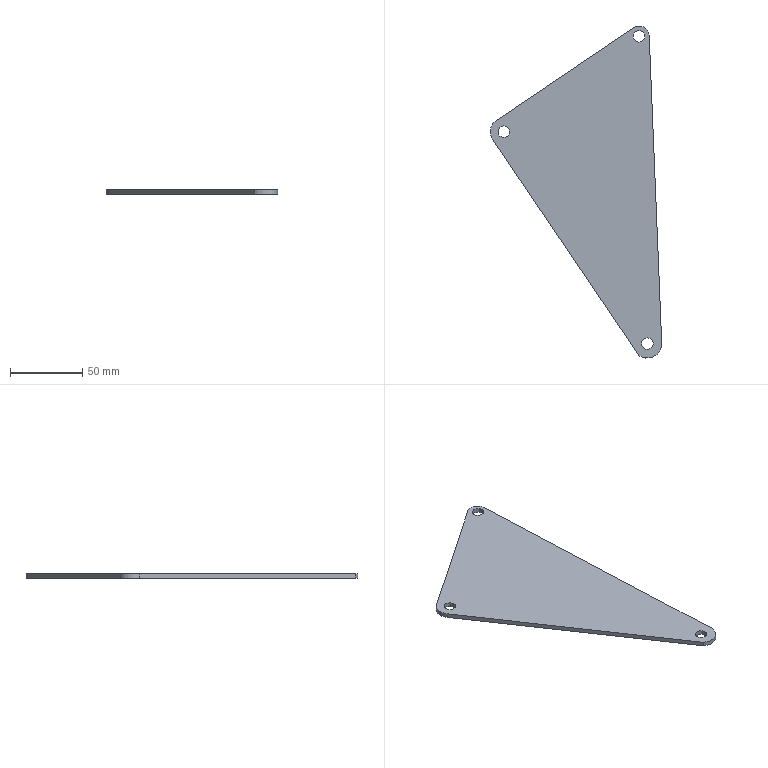Component | SolidWorks | gen par_a-2 | 1 solid | 15 faces | box 118.62 x 229.7 x 3 mm | volume 43932 mm3 | cylinder 10 | plane 5 | commonest cylinder face diameters 8 x6 14.196 x2 20 x1 18.711 x1
STEP:
#1=CARTESIAN_POINT('',(8.88,0.8832,7.243));
#2=VERTEX_POINT('',#1);
#3=CARTESIAN_POINT('',(9.14,1.06,7.243));
#4=VERTEX_POINT('',#3);
#5=CARTESIAN_POINT('',(9.01,0.9715,7.243));
#6=DIRECTION('',(-0.,0.,1.));
#7=DIRECTION('',(0.8279,0.5608,0.));
#8=AXIS2_PLACEMENT_3D('',#5,#6,#7);
#9=CIRCLE('',#8,0.1575);
#10=EDGE_CURVE('',#2,#4,#9,.T.);
#11=ORIENTED_EDGE('',*,*,#10,.F.);
#12=CARTESIAN_POINT('',(8.88,0.8832,7.361));
#13=VERTEX_POINT('',#12);
#14=CARTESIAN_POINT('',(8.88,0.8832,7.243));
#15=DIRECTION('',(-0.,0.,1.));
#16=VECTOR('',#15,39.37);
#17=LINE('',#14,#16);
#18=EDGE_CURVE('',#2,#13,#17,.T.);
#19=ORIENTED_EDGE('',*,*,#18,.T.);
#20=CARTESIAN_POINT('',(9.14,1.06,7.361));
#21=VERTEX_POINT('',#20);
#22=CARTESIAN_POINT('',(9.01,0.9715,7.361));
#23=DIRECTION('',(-0.,0.,1.));
#24=DIRECTION('',(0.8279,0.5608,0.));
#25=AXIS2_PLACEMENT_3D('',#22,#23,#24);
#26=CIRCLE('',#25,0.1575);
#27=EDGE_CURVE('',#13,#21,#26,.T.);
#28=ORIENTED_EDGE('',*,*,#27,.T.);
#29=CARTESIAN_POINT('',(9.14,1.06,7.243));
#30=DIRECTION('',(-0.,0.,1.));
#31=VECTOR('',#30,39.37);
#32=LINE('',#29,#31);
#33=EDGE_CURVE('',#4,#21,#32,.T.);
#34=ORIENTED_EDGE('',*,*,#33,.F.);
#35=EDGE_LOOP('',(#11,#19,#28,#34));
#36=FACE_OUTER_BOUND('',#35,.T.);
#37=CARTESIAN_POINT('',(9.01,0.9715,7.243));
#38=DIRECTION('',(-0.,0.,1.));
#39=DIRECTION('',(0.8279,0.5608,0.));
#40=AXIS2_PLACEMENT_3D('',#37,#38,#39);
#41=CYLINDRICAL_SURFACE('',#40,0.1575);
#42=ADVANCED_FACE('',(#36),#41,.F.);
#43=CARTESIAN_POINT('',(8.652,9.253,7.243));
#44=VERTEX_POINT('',#43);
#45=CARTESIAN_POINT('',(8.913,9.43,7.243));
#46=VERTEX_POINT('',#45);
#47=CARTESIAN_POINT('',(8.783,9.342,7.243));
#48=DIRECTION('',(-0.,0.,1.));
#49=DIRECTION('',(0.8279,0.5608,0.));
#50=AXIS2_PLACEMENT_3D('',#47,#48,#49);
#51=CIRCLE('',#50,0.1575);
#52=EDGE_CURVE('',#44,#46,#51,.T.);
#53=ORIENTED_EDGE('',*,*,#52,.F.);
#54=CARTESIAN_POINT('',(8.652,9.253,7.361));
#55=VERTEX_POINT('',#54);
#56=CARTESIAN_POINT('',(8.652,9.253,7.243));
#57=DIRECTION('',(-0.,0.,1.));
#58=VECTOR('',#57,39.37);
#59=LINE('',#56,#58);
#60=EDGE_CURVE('',#44,#55,#59,.T.);
#61=ORIENTED_EDGE('',*,*,#60,.T.);
#62=CARTESIAN_POINT('',(8.913,9.43,7.361));
#63=VERTEX_POINT('',#62);
#64=CARTESIAN_POINT('',(8.783,9.342,7.361));
#65=DIRECTION('',(-0.,0.,1.));
#66=DIRECTION('',(0.8279,0.5608,0.));
#67=AXIS2_PLACEMENT_3D('',#64,#65,#66);
#68=CIRCLE('',#67,0.1575);
#69=EDGE_CURVE('',#55,#63,#68,.T.);
#70=ORIENTED_EDGE('',*,*,#69,.T.);
#71=CARTESIAN_POINT('',(8.913,9.43,7.243));
#72=DIRECTION('',(-0.,0.,1.));
#73=VECTOR('',#72,39.37);
#74=LINE('',#71,#73);
#75=EDGE_CURVE('',#46,#63,#74,.T.);
#76=ORIENTED_EDGE('',*,*,#75,.F.);
#77=EDGE_LOOP('',(#53,#61,#70,#76));
#78=FACE_OUTER_BOUND('',#77,.T.);
#79=CARTESIAN_POINT('',(8.783,9.342,7.243));
#80=DIRECTION('',(-0.,0.,1.));
#81=DIRECTION('',(0.8279,0.5608,0.));
#82=AXIS2_PLACEMENT_3D('',#79,#80,#81);
#83=CYLINDRICAL_SURFACE('',#82,0.1575);
#84=ADVANCED_FACE('',(#78),#83,.F.);
#85=CARTESIAN_POINT('',(4.971,6.653,7.243));
#86=VERTEX_POINT('',#85);
#87=CARTESIAN_POINT('',(5.232,6.829,7.243));
#88=VERTEX_POINT('',#87);
#89=CARTESIAN_POINT('',(5.102,6.741,7.243));
#90=DIRECTION('',(-0.,0.,1.));
#91=DIRECTION('',(0.8279,0.5608,0.));
#92=AXIS2_PLACEMENT_3D('',#89,#90,#91);
#93=CIRCLE('',#92,0.1575);
#94=EDGE_CURVE('',#86,#88,#93,.T.);
#95=ORIENTED_EDGE('',*,*,#94,.F.);
#96=CARTESIAN_POINT('',(4.971,6.653,7.361));
#97=VERTEX_POINT('',#96);
#98=CARTESIAN_POINT('',(4.971,6.653,7.243));
#99=DIRECTION('',(-0.,0.,1.));
#100=VECTOR('',#99,39.37);
#101=LINE('',#98,#100);
#102=EDGE_CURVE('',#86,#97,#101,.T.);
#103=ORIENTED_EDGE('',*,*,#102,.T.);
#104=CARTESIAN_POINT('',(5.232,6.829,7.361));
#105=VERTEX_POINT('',#104);
#106=CARTESIAN_POINT('',(5.102,6.741,7.361));
#107=DIRECTION('',(-0.,0.,1.));
#108=DIRECTION('',(0.8279,0.5608,0.));
#109=AXIS2_PLACEMENT_3D('',#106,#107,#108);
#110=CIRCLE('',#109,0.1575);
#111=EDGE_CURVE('',#97,#105,#110,.T.);
#112=ORIENTED_EDGE('',*,*,#111,.T.);
#113=CARTESIAN_POINT('',(5.232,6.829,7.243));
#114=DIRECTION('',(-0.,0.,1.));
#115=VECTOR('',#114,39.37);
#116=LINE('',#113,#115);
#117=EDGE_CURVE('',#88,#105,#116,.T.);
#118=ORIENTED_EDGE('',*,*,#117,.F.);
#119=EDGE_LOOP('',(#95,#103,#112,#118));
#120=FACE_OUTER_BOUND('',#119,.T.);
#121=CARTESIAN_POINT('',(5.102,6.741,7.243));
#122=DIRECTION('',(-0.,0.,1.));
#123=DIRECTION('',(0.8279,0.5608,0.));
#124=AXIS2_PLACEMENT_3D('',#121,#122,#123);
#125=CYLINDRICAL_SURFACE('',#124,0.1575);
#126=ADVANCED_FACE('',(#120),#125,.F.);
#127=CARTESIAN_POINT('',(9.062,9.353,7.243));
#128=VERTEX_POINT('',#127);
#129=CARTESIAN_POINT('',(9.014,9.498,7.243));
#130=VERTEX_POINT('',#129);
#131=CARTESIAN_POINT('',(8.783,9.342,7.243));
#132=DIRECTION('',(-0.,0.,1.));
#133=DIRECTION('',(0.8279,0.5608,0.));
#134=AXIS2_PLACEMENT_3D('',#131,#132,#133);
#135=CIRCLE('',#134,0.2795);
#136=EDGE_CURVE('',#128,#130,#135,.T.);
#137=ORIENTED_EDGE('',*,*,#136,.T.);
#138=CARTESIAN_POINT('',(9.014,9.498,7.361));
#139=VERTEX_POINT('',#138);
#140=CARTESIAN_POINT('',(9.014,9.498,7.243));
#141=DIRECTION('',(-0.,0.,1.));
#142=VECTOR('',#141,39.37);
#143=LINE('',#140,#142);
#144=EDGE_CURVE('',#130,#139,#143,.T.);
#145=ORIENTED_EDGE('',*,*,#144,.T.);
#146=CARTESIAN_POINT('',(9.062,9.353,7.361));
#147=VERTEX_POINT('',#146);
#148=CARTESIAN_POINT('',(8.783,9.342,7.361));
#149=DIRECTION('',(-0.,0.,1.));
#150=DIRECTION('',(0.8279,0.5608,0.));
#151=AXIS2_PLACEMENT_3D('',#148,#149,#150);
#152=CIRCLE('',#151,0.2795);
#153=EDGE_CURVE('',#147,#139,#152,.T.);
#154=ORIENTED_EDGE('',*,*,#153,.F.);
#155=CARTESIAN_POINT('',(9.062,9.353,7.243));
#156=DIRECTION('',(-0.,0.,1.));
#157=VECTOR('',#156,39.37);
#158=LINE('',#155,#157);
#159=EDGE_CURVE('',#128,#147,#158,.T.);
#160=ORIENTED_EDGE('',*,*,#159,.F.);
#161=EDGE_LOOP('',(#137,#145,#154,#160));
#162=FACE_OUTER_BOUND('',#161,.T.);
#163=CARTESIAN_POINT('',(8.783,9.342,7.243));
#164=DIRECTION('',(-0.,0.,1.));
#165=DIRECTION('',(0.8279,0.5608,0.));
#166=AXIS2_PLACEMENT_3D('',#163,#164,#165);
#167=CYLINDRICAL_SURFACE('',#166,0.2795);
#168=ADVANCED_FACE('',(#162),#167,.T.);
#169=CARTESIAN_POINT('',(8.783,0.6498,7.361));
#170=VERTEX_POINT('',#169);
#171=CARTESIAN_POINT('',(9.403,0.9876,7.361));
#172=VERTEX_POINT('',#171);
#173=CARTESIAN_POINT('',(9.01,0.9715,7.361));
#174=DIRECTION('',(-0.,0.,1.));
#175=DIRECTION('',(0.8279,0.5608,0.));
#176=AXIS2_PLACEMENT_3D('',#173,#174,#175);
#177=CIRCLE('',#176,0.3937);
#178=EDGE_CURVE('',#170,#172,#177,.T.);
#179=ORIENTED_EDGE('',*,*,#178,.F.);
#180=CARTESIAN_POINT('',(8.783,0.6498,7.243));
#181=VERTEX_POINT('',#180);
#182=CARTESIAN_POINT('',(8.783,0.6498,7.243));
#183=DIRECTION('',(-0.,0.,1.));
#184=VECTOR('',#183,39.37);
#185=LINE('',#182,#184);
#186=EDGE_CURVE('',#181,#170,#185,.T.);
#187=ORIENTED_EDGE('',*,*,#186,.F.);
#188=CARTESIAN_POINT('',(9.403,0.9876,7.243));
#189=VERTEX_POINT('',#188);
#190=CARTESIAN_POINT('',(9.01,0.9715,7.243));
#191=DIRECTION('',(-0.,0.,1.));
#192=DIRECTION('',(0.8279,0.5608,0.));
#193=AXIS2_PLACEMENT_3D('',#190,#191,#192);
#194=CIRCLE('',#193,0.3937);
#195=EDGE_CURVE('',#181,#189,#194,.T.);
#196=ORIENTED_EDGE('',*,*,#195,.T.);
#197=CARTESIAN_POINT('',(9.403,0.9876,7.243));
#198=DIRECTION('',(-0.,0.,1.));
#199=VECTOR('',#198,39.37);
#200=LINE('',#197,#199);
#201=EDGE_CURVE('',#189,#172,#200,.T.);
#202=ORIENTED_EDGE('',*,*,#201,.T.);
#203=EDGE_LOOP('',(#179,#187,#196,#202));
#204=FACE_OUTER_BOUND('',#203,.T.);
#205=CARTESIAN_POINT('',(9.01,0.9715,7.243));
#206=DIRECTION('',(-0.,0.,1.));
#207=DIRECTION('',(0.8279,0.5608,0.));
#208=AXIS2_PLACEMENT_3D('',#205,#206,#207);
#209=CYLINDRICAL_SURFACE('',#208,0.3937);
#210=ADVANCED_FACE('',(#204),#209,.T.);
#211=CARTESIAN_POINT('',(4.797,6.534,7.361));
#212=VERTEX_POINT('',#211);
#213=CARTESIAN_POINT('',(8.783,0.6498,7.361));
#214=DIRECTION('',(0.5608,-0.8279,0.));
#215=VECTOR('',#214,39.37);
#216=LINE('',#213,#215);
#217=EDGE_CURVE('',#212,#170,#216,.T.);
#218=ORIENTED_EDGE('',*,*,#217,.F.);
#219=CARTESIAN_POINT('',(4.797,6.534,7.243));
#220=VERTEX_POINT('',#219);
#221=CARTESIAN_POINT('',(4.797,6.534,7.243));
#222=DIRECTION('',(-0.,0.,1.));
#223=VECTOR('',#222,39.37);
#224=LINE('',#221,#223);
#225=EDGE_CURVE('',#220,#212,#224,.T.);
#226=ORIENTED_EDGE('',*,*,#225,.F.);
#227=CARTESIAN_POINT('',(8.783,0.6498,7.243));
#228=DIRECTION('',(0.5608,-0.8279,0.));
#229=VECTOR('',#228,39.37);
#230=LINE('',#227,#229);
#231=EDGE_CURVE('',#220,#181,#230,.T.);
#232=ORIENTED_EDGE('',*,*,#231,.T.);
#233=ORIENTED_EDGE('',*,*,#186,.T.);
#234=EDGE_LOOP('',(#218,#226,#232,#233));
#235=FACE_OUTER_BOUND('',#234,.T.);
#236=CARTESIAN_POINT('',(8.783,0.6498,7.243));
#237=DIRECTION('',(-0.8279,-0.5608,-0.));
#238=DIRECTION('',(-0.,0.,1.));
#239=AXIS2_PLACEMENT_3D('',#236,#237,#238);
#240=PLANE('',#239);
#241=ADVANCED_FACE('',(#235),#240,.T.);
#242=CARTESIAN_POINT('',(4.895,7.046,7.361));
#243=VERTEX_POINT('',#242);
#244=CARTESIAN_POINT('',(5.102,6.741,7.361));
#245=DIRECTION('',(-0.,0.,1.));
#246=DIRECTION('',(-0.8279,-0.5608,0.));
#247=AXIS2_PLACEMENT_3D('',#244,#245,#246);
#248=CIRCLE('',#247,0.3683);
#249=EDGE_CURVE('',#243,#212,#248,.T.);
#250=ORIENTED_EDGE('',*,*,#249,.F.);
#251=CARTESIAN_POINT('',(4.895,7.046,7.243));
#252=VERTEX_POINT('',#251);
#253=CARTESIAN_POINT('',(4.895,7.046,7.243));
#254=DIRECTION('',(-0.,0.,1.));
#255=VECTOR('',#254,39.37);
#256=LINE('',#253,#255);
#257=EDGE_CURVE('',#252,#243,#256,.T.);
#258=ORIENTED_EDGE('',*,*,#257,.F.);
#259=CARTESIAN_POINT('',(5.102,6.741,7.243));
#260=DIRECTION('',(-0.,0.,1.));
#261=DIRECTION('',(-0.8279,-0.5608,0.));
#262=AXIS2_PLACEMENT_3D('',#259,#260,#261);
#263=CIRCLE('',#262,0.3683);
#264=EDGE_CURVE('',#252,#220,#263,.T.);
#265=ORIENTED_EDGE('',*,*,#264,.T.);
#266=ORIENTED_EDGE('',*,*,#225,.T.);
#267=EDGE_LOOP('',(#250,#258,#265,#266));
#268=FACE_OUTER_BOUND('',#267,.T.);
#269=CARTESIAN_POINT('',(5.102,6.741,7.243));
#270=DIRECTION('',(-0.,0.,1.));
#271=DIRECTION('',(0.8279,0.5608,0.));
#272=AXIS2_PLACEMENT_3D('',#269,#270,#271);
#273=CYLINDRICAL_SURFACE('',#272,0.3683);
#274=ADVANCED_FACE('',(#268),#273,.T.);
#275=CARTESIAN_POINT('',(8.626,9.573,7.361));
#276=VERTEX_POINT('',#275);
#277=CARTESIAN_POINT('',(4.895,7.046,7.361));
#278=DIRECTION('',(-0.8279,-0.5608,-0.));
#279=VECTOR('',#278,39.37);
#280=LINE('',#277,#279);
#281=EDGE_CURVE('',#276,#243,#280,.T.);
#282=ORIENTED_EDGE('',*,*,#281,.F.);
#283=CARTESIAN_POINT('',(8.626,9.573,7.243));
#284=VERTEX_POINT('',#283);
#285=CARTESIAN_POINT('',(8.626,9.573,7.243));
#286=DIRECTION('',(-0.,0.,1.));
#287=VECTOR('',#286,39.37);
#288=LINE('',#285,#287);
#289=EDGE_CURVE('',#284,#276,#288,.T.);
#290=ORIENTED_EDGE('',*,*,#289,.F.);
#291=CARTESIAN_POINT('',(4.895,7.046,7.243));
#292=DIRECTION('',(-0.8279,-0.5608,-0.));
#293=VECTOR('',#292,39.37);
#294=LINE('',#291,#293);
#295=EDGE_CURVE('',#284,#252,#294,.T.);
#296=ORIENTED_EDGE('',*,*,#295,.T.);
#297=ORIENTED_EDGE('',*,*,#257,.T.);
#298=EDGE_LOOP('',(#282,#290,#296,#297));
#299=FACE_OUTER_BOUND('',#298,.T.);
#300=CARTESIAN_POINT('',(4.895,7.046,7.243));
#301=DIRECTION('',(-0.5608,0.8279,-0.));
#302=DIRECTION('',(-0.8279,-0.5608,-0.));
#303=AXIS2_PLACEMENT_3D('',#300,#301,#302);
#304=PLANE('',#303);
#305=ADVANCED_FACE('',(#299),#304,.T.);
#306=ORIENTED_EDGE('',*,*,#144,.F.);
#307=CARTESIAN_POINT('',(8.783,9.342,7.243));
#308=DIRECTION('',(-0.,0.,1.));
#309=DIRECTION('',(0.8279,0.5608,0.));
#310=AXIS2_PLACEMENT_3D('',#307,#308,#309);
#311=CIRCLE('',#310,0.2795);
#312=EDGE_CURVE('',#130,#284,#311,.T.);
#313=ORIENTED_EDGE('',*,*,#312,.T.);
#314=ORIENTED_EDGE('',*,*,#289,.T.);
#315=CARTESIAN_POINT('',(8.783,9.342,7.361));
#316=DIRECTION('',(-0.,0.,1.));
#317=DIRECTION('',(0.8279,0.5608,0.));
#318=AXIS2_PLACEMENT_3D('',#315,#316,#317);
#319=CIRCLE('',#318,0.2795);
#320=EDGE_CURVE('',#139,#276,#319,.T.);
#321=ORIENTED_EDGE('',*,*,#320,.F.);
#322=EDGE_LOOP('',(#306,#313,#314,#321));
#323=FACE_OUTER_BOUND('',#322,.T.);
#324=CARTESIAN_POINT('',(8.783,9.342,7.243));
#325=DIRECTION('',(-0.,0.,1.));
#326=DIRECTION('',(0.8279,0.5608,0.));
#327=AXIS2_PLACEMENT_3D('',#324,#325,#326);
#328=CYLINDRICAL_SURFACE('',#327,0.2795);
#329=ADVANCED_FACE('',(#323),#328,.T.);
#330=CARTESIAN_POINT('',(9.403,0.9876,7.361));
#331=DIRECTION('',(-0.04078,0.9992,-0.));
#332=VECTOR('',#331,39.37);
#333=LINE('',#330,#332);
#334=EDGE_CURVE('',#172,#147,#333,.T.);
#335=ORIENTED_EDGE('',*,*,#334,.F.);
#336=ORIENTED_EDGE('',*,*,#201,.F.);
#337=CARTESIAN_POINT('',(9.403,0.9876,7.243));
#338=DIRECTION('',(-0.04078,0.9992,-0.));
#339=VECTOR('',#338,39.37);
#340=LINE('',#337,#339);
#341=EDGE_CURVE('',#189,#128,#340,.T.);
#342=ORIENTED_EDGE('',*,*,#341,.T.);
#343=ORIENTED_EDGE('',*,*,#159,.T.);
#344=EDGE_LOOP('',(#335,#336,#342,#343));
#345=FACE_OUTER_BOUND('',#344,.T.);
#346=CARTESIAN_POINT('',(9.403,0.9876,7.243));
#347=DIRECTION('',(0.9992,0.04078,0.));
#348=DIRECTION('',(-0.04078,0.9992,-0.));
#349=AXIS2_PLACEMENT_3D('',#346,#347,#348);
#350=PLANE('',#349);
#351=ADVANCED_FACE('',(#345),#350,.T.);
#352=CARTESIAN_POINT('',(9.01,0.9715,7.243));
#353=DIRECTION('',(-0.,0.,1.));
#354=DIRECTION('',(0.8279,0.5608,0.));
#355=AXIS2_PLACEMENT_3D('',#352,#353,#354);
#356=CIRCLE('',#355,0.1575);
#357=EDGE_CURVE('',#4,#2,#356,.T.);
#358=ORIENTED_EDGE('',*,*,#357,.T.);
#359=ORIENTED_EDGE('',*,*,#10,.T.);
#360=EDGE_LOOP('',(#358,#359));
#361=FACE_BOUND('',#360,.T.);
#362=CARTESIAN_POINT('',(8.783,9.342,7.243));
#363=DIRECTION('',(-0.,0.,1.));
#364=DIRECTION('',(0.8279,0.5608,0.));
#365=AXIS2_PLACEMENT_3D('',#362,#363,#364);
#366=CIRCLE('',#365,0.1575);
#367=EDGE_CURVE('',#46,#44,#366,.T.);
#368=ORIENTED_EDGE('',*,*,#367,.T.);
#369=ORIENTED_EDGE('',*,*,#52,.T.);
#370=EDGE_LOOP('',(#368,#369));
#371=FACE_BOUND('',#370,.T.);
#372=CARTESIAN_POINT('',(5.102,6.741,7.243));
#373=DIRECTION('',(-0.,0.,1.));
#374=DIRECTION('',(0.8279,0.5608,0.));
#375=AXIS2_PLACEMENT_3D('',#372,#373,#374);
#376=CIRCLE('',#375,0.1575);
#377=EDGE_CURVE('',#88,#86,#376,.T.);
#378=ORIENTED_EDGE('',*,*,#377,.T.);
#379=ORIENTED_EDGE('',*,*,#94,.T.);
#380=EDGE_LOOP('',(#378,#379));
#381=FACE_BOUND('',#380,.T.);
#382=ORIENTED_EDGE('',*,*,#195,.F.);
#383=ORIENTED_EDGE('',*,*,#231,.F.);
#384=ORIENTED_EDGE('',*,*,#264,.F.);
#385=ORIENTED_EDGE('',*,*,#295,.F.);
#386=ORIENTED_EDGE('',*,*,#312,.F.);
#387=ORIENTED_EDGE('',*,*,#136,.F.);
#388=ORIENTED_EDGE('',*,*,#341,.F.);
#389=EDGE_LOOP('',(#382,#383,#384,#385,#386,#387,#388));
#390=FACE_OUTER_BOUND('',#389,.T.);
#391=CARTESIAN_POINT('',(9.01,0.9715,7.243));
#392=DIRECTION('',(-0.,0.,1.));
#393=DIRECTION('',(0.8279,0.5608,0.));
#394=AXIS2_PLACEMENT_3D('',#391,#392,#393);
#395=PLANE('',#394);
#396=ADVANCED_FACE('',(#361,#371,#381,#390),#395,.F.);
#397=CARTESIAN_POINT('',(9.01,0.9715,7.361));
#398=DIRECTION('',(-0.,0.,1.));
#399=DIRECTION('',(0.8279,0.5608,0.));
#400=AXIS2_PLACEMENT_3D('',#397,#398,#399);
#401=CIRCLE('',#400,0.1575);
#402=EDGE_CURVE('',#21,#13,#401,.T.);
#403=ORIENTED_EDGE('',*,*,#402,.F.);
#404=ORIENTED_EDGE('',*,*,#27,.F.);
#405=EDGE_LOOP('',(#403,#404));
#406=FACE_BOUND('',#405,.T.);
#407=CARTESIAN_POINT('',(8.783,9.342,7.361));
#408=DIRECTION('',(-0.,0.,1.));
#409=DIRECTION('',(0.8279,0.5608,0.));
#410=AXIS2_PLACEMENT_3D('',#407,#408,#409);
#411=CIRCLE('',#410,0.1575);
#412=EDGE_CURVE('',#63,#55,#411,.T.);
#413=ORIENTED_EDGE('',*,*,#412,.F.);
#414=ORIENTED_EDGE('',*,*,#69,.F.);
#415=EDGE_LOOP('',(#413,#414));
#416=FACE_BOUND('',#415,.T.);
#417=CARTESIAN_POINT('',(5.102,6.741,7.361));
#418=DIRECTION('',(-0.,0.,1.));
#419=DIRECTION('',(0.8279,0.5608,0.));
#420=AXIS2_PLACEMENT_3D('',#417,#418,#419);
#421=CIRCLE('',#420,0.1575);
#422=EDGE_CURVE('',#105,#97,#421,.T.);
#423=ORIENTED_EDGE('',*,*,#422,.F.);
#424=ORIENTED_EDGE('',*,*,#111,.F.);
#425=EDGE_LOOP('',(#423,#424));
#426=FACE_BOUND('',#425,.T.);
#427=ORIENTED_EDGE('',*,*,#178,.T.);
#428=ORIENTED_EDGE('',*,*,#334,.T.);
#429=ORIENTED_EDGE('',*,*,#153,.T.);
#430=ORIENTED_EDGE('',*,*,#320,.T.);
#431=ORIENTED_EDGE('',*,*,#281,.T.);
#432=ORIENTED_EDGE('',*,*,#249,.T.);
#433=ORIENTED_EDGE('',*,*,#217,.T.);
#434=EDGE_LOOP('',(#427,#428,#429,#430,#431,#432,#433));
#435=FACE_OUTER_BOUND('',#434,.T.);
#436=CARTESIAN_POINT('',(9.01,0.9715,7.361));
#437=DIRECTION('',(-0.,0.,1.));
#438=DIRECTION('',(0.8279,0.5608,0.));
#439=AXIS2_PLACEMENT_3D('',#436,#437,#438);
#440=PLANE('',#439);
#441=ADVANCED_FACE('',(#406,#416,#426,#435),#440,.T.);
#442=ORIENTED_EDGE('',*,*,#102,.F.);
#443=ORIENTED_EDGE('',*,*,#377,.F.);
#444=ORIENTED_EDGE('',*,*,#117,.T.);
#445=ORIENTED_EDGE('',*,*,#422,.T.);
#446=EDGE_LOOP('',(#442,#443,#444,#445));
#447=FACE_OUTER_BOUND('',#446,.T.);
#448=CARTESIAN_POINT('',(5.102,6.741,7.243));
#449=DIRECTION('',(-0.,0.,1.));
#450=DIRECTION('',(0.8279,0.5608,0.));
#451=AXIS2_PLACEMENT_3D('',#448,#449,#450);
#452=CYLINDRICAL_SURFACE('',#451,0.1575);
#453=ADVANCED_FACE('',(#447),#452,.F.);
#454=ORIENTED_EDGE('',*,*,#60,.F.);
#455=ORIENTED_EDGE('',*,*,#367,.F.);
#456=ORIENTED_EDGE('',*,*,#75,.T.);
#457=ORIENTED_EDGE('',*,*,#412,.T.);
#458=EDGE_LOOP('',(#454,#455,#456,#457));
#459=FACE_OUTER_BOUND('',#458,.T.);
#460=CARTESIAN_POINT('',(8.783,9.342,7.243));
#461=DIRECTION('',(-0.,0.,1.));
#462=DIRECTION('',(0.8279,0.5608,0.));
#463=AXIS2_PLACEMENT_3D('',#460,#461,#462);
#464=CYLINDRICAL_SURFACE('',#463,0.1575);
#465=ADVANCED_FACE('',(#459),#464,.F.);
#466=ORIENTED_EDGE('',*,*,#18,.F.);
#467=ORIENTED_EDGE('',*,*,#357,.F.);
#468=ORIENTED_EDGE('',*,*,#33,.T.);
#469=ORIENTED_EDGE('',*,*,#402,.T.);
#470=EDGE_LOOP('',(#466,#467,#468,#469));
#471=FACE_OUTER_BOUND('',#470,.T.);
#472=CARTESIAN_POINT('',(9.01,0.9715,7.243));
#473=DIRECTION('',(-0.,0.,1.));
#474=DIRECTION('',(0.8279,0.5608,0.));
#475=AXIS2_PLACEMENT_3D('',#472,#473,#474);
#476=CYLINDRICAL_SURFACE('',#475,0.1575);
#477=ADVANCED_FACE('',(#471),#476,.F.);
#478=CLOSED_SHELL('',(#42,#84,#126,#168,#210,#241,#274,#305,#329,#351,#396,#441,#453,#465,#477));
#479=MANIFOLD_SOLID_BREP('',#478);
#480=CARTESIAN_POINT('',(0.,0.,0.));
#481=DIRECTION('',(0.,0.,1.));
#482=DIRECTION('',(1.,0.,0.));
#483=AXIS2_PLACEMENT_3D('',#480,#481,#482);
#484=(LENGTH_UNIT()NAMED_UNIT(*)SI_UNIT($,.METRE.));
#485=LENGTH_MEASURE_WITH_UNIT(LENGTH_MEASURE(0.0254),#484);
#486=DIMENSIONAL_EXPONENTS(1.,0.,0.,0.,0.,0.,0.);
#487=(CONVERSION_BASED_UNIT('',#485)LENGTH_UNIT()NAMED_UNIT(#486));
#488=UNCERTAINTY_MEASURE_WITH_UNIT(LENGTH_MEASURE(0.00001),#487,'','');
#489=(NAMED_UNIT(*)PLANE_ANGLE_UNIT()SI_UNIT($,.RADIAN.));
#490=(NAMED_UNIT(*)SI_UNIT($,.STERADIAN.)SOLID_ANGLE_UNIT());
#491=(GEOMETRIC_REPRESENTATION_CONTEXT(3)GLOBAL_UNCERTAINTY_ASSIGNED_CONTEXT((#488))GLOBAL_UNIT_ASSIGNED_CONTEXT((#487,#489,#490))REPRESENTATION_CONTEXT('',''));
#492=ADVANCED_BREP_SHAPE_REPRESENTATION('',(#479,#483),#491);
#493=COLOUR_RGB('',0.7922,0.8196,0.9333);
#494=FILL_AREA_STYLE_COLOUR('',#493);
#495=FILL_AREA_STYLE('',(#494));
#496=SURFACE_STYLE_FILL_AREA(#495);
#497=SURFACE_SIDE_STYLE('',(#496));
#498=SURFACE_STYLE_USAGE(.BOTH.,#497);
#499=PRESENTATION_STYLE_ASSIGNMENT((#498));
#500=STYLED_ITEM('',(#499),#479);
#501=(LENGTH_UNIT()NAMED_UNIT(*)SI_UNIT($,.METRE.));
#502=LENGTH_MEASURE_WITH_UNIT(LENGTH_MEASURE(0.0254),#501);
#503=DIMENSIONAL_EXPONENTS(1.,0.,0.,0.,0.,0.,0.);
#504=(CONVERSION_BASED_UNIT('',#502)LENGTH_UNIT()NAMED_UNIT(#503));
#505=UNCERTAINTY_MEASURE_WITH_UNIT(LENGTH_MEASURE(0.00001),#504,'','');
#506=(NAMED_UNIT(*)PLANE_ANGLE_UNIT()SI_UNIT($,.RADIAN.));
#507=(NAMED_UNIT(*)SI_UNIT($,.STERADIAN.)SOLID_ANGLE_UNIT());
#508=(GEOMETRIC_REPRESENTATION_CONTEXT(3)GLOBAL_UNCERTAINTY_ASSIGNED_CONTEXT((#505))GLOBAL_UNIT_ASSIGNED_CONTEXT((#504,#506,#507))REPRESENTATION_CONTEXT('',''));
#509=MECHANICAL_DESIGN_GEOMETRIC_PRESENTATION_REPRESENTATION('',(#500),#508);
#510=PRESENTATION_LAYER_ASSIGNMENT('','',(#500));